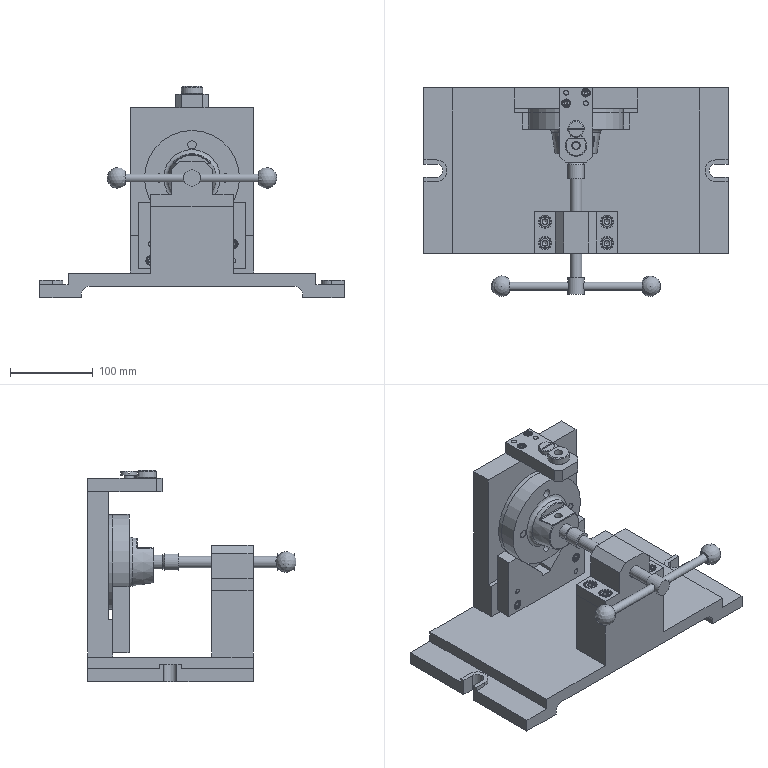Assembly | NX | mm | 27 component files | 27 solids | 499 faces | box 368 x 252.5 x 256 mm | volume 3203804 mm3 | plane 256 | cone 118 | cylinder 98 | torus 19 | sphere 4 | spline 4 | commonest cylinder face diameters 6 x15 10 x15 8 x12 15 x6 20 x5 9 x5 7.76 x4 13 x4
Bill of materials:
GB-T70.1-2000,M8x20 | 4 |  | Hexagon Socket Head Cap Screw, GB-T 70.1-2000,M8x20
unnamed part 1 | 1 |  | Long, slender cylindrical pin with a short, smaller-diameter stepped journal at each end.
unnamed part 2 | 1 |  | Cylindrical pin with a larger-diameter head at one end. A transverse through-hole crosses the head. The opposite end steps down to a short smaller-diameter journal.
unnamed part 3 | 1 |  | Stepped shaft: a hexagonal section at one end, a larger cylindrical collar in the middle, and a smaller cylindrical spigot with a chamfered end.
unnamed part 4 | 1 |  | Thick-walled cylindrical sleeve with a central bore and an outer chamfer at one end.
GB-T119.1-2000,10x30 | 1 |  | Parallel Pin, GB-T 119.1-2000,10x30
unnamed part 5 | 1 |  | Shouldered pin with a slotted head: a chamfered disc head with a straight slot, a cylindrical shoulder, a narrow neck or undercut, and a chamfered cylindrical pilot end.
unnamed part 6 | 1 |  | Pillow-block-style bracket: a rectangular base plate with a raised central block. The block has chamfered upper corners and one horizontal through-bore.
unnamed part 7 | 1 |  | Flanged bushing: a cylindrical body with a larger chamfered flange at one end and a central through-bore. The flange has a flat or notch cut on one side.
GB-T119.1-2000,6x22 | 2 |  | Parallel Pin, GB-T 119.1-2000,6x22
unnamed part 8 | 2 |  | Sphere with uniform, ball-like form.
unnamed part 9 | 1 |  | Plain cylindrical tube or spacer ring with a concentric through-bore and square ends.
unnamed part 10 | 1 |  | Rectangular plate with a symmetric V-shaped notch cut into one long edge. A small rectangular slot sits at the bottom of the V. The plate has four through-holes near its ends.
unnamed part 11 | 1 |  | Circular flange with a tapered hub on one side. The hub has a flat face with a cross-hole and ends in a small cylindrical spigot. The opposite face has a central circular recess.
unnamed part 12 | 1 |  | Rectangular plate with two chamfered corners at one end, one large through-hole, one medium hole, and four small holes grouped at the opposite end.
GB-T119.1-2000,6x26 | 2 |  | Parallel Pin, GB-T 119.1-2000,6x26
unnamed part 13 | 1 |  | Prismatic, machined-looking base plate with a rectangular block standing near one end and a tall upright plate near the other. The base has thinner stepped flanges at both ends, each with an open-ended U-slot, and a wide shallow relief with rounded ends across the underside. The upright plate has a slightly raised or recessed circular face carrying small holes, a raised strip along its lower edge with holes, and small holes on its top edge. The block has holes on its top face.
GB-T70.1-2000,M5x16 | 2 |  | Hexagon Socket Head Cap Screw, GB-T 70.1-2000,M5x16
GB-T70.1-2000,M6x20 | 2 |  | Hexagon Socket Head Cap Screw, GB-T 70.1-2000,M6x20
Mates:
1. fix | fixture_body 1 component
2. concentric | base 1 edge | fixture_body 1 edge
3. touch align | fixed_v_block 1 face | base 1 face
4. touch align | fixed_v_block 1 face | base 1 face
5. touch align | fixed_v_block 1 face | base 1 face
6. concentric | bushing 1 edge | drill_template 1 edge
7. concentric | drill_bushing 1 edge | bushing 1 edge
8. concentric | drill_bushing_screw 1 edge | drill_template 1 edge
9. touch align | drill_template 1 face | fixture_body 1 face
10. center | drill_template 1 face | drill_template 1 face | fixture_body 1 face | fixture_body 1 face
11. touch align | drill_template 1 face | fixture_body 1 face
12. touch align | screw_rod 1 face | fixed_bracket 1 face
13. concentric | rubber_pad 1 edge | screw_rod 1 edge
14. touch align | rubber_pad 1 face | base 1 face
15. touch align | handle 1 face | screw_rod 1 face
16. center | handle 1 face | handle 1 face | fixed_bracket 1 face | fixed_bracket 1 face
17. concentric | handle_1 2 edge | handle 1 edge
18. concentric | handle_1 1 edge | handle 1 edge
19. concentric | diamond_locating_pin 1 edge | fixture_body 1 edge
20. concentric | GB-T70_1-2000_M8x20 1 edge | fixed_bracket 1 edge
21. concentric | GB-T70_1-2000_M8x20 2 edge | fixed_bracket 1 edge
22. concentric | GB-T70_1-2000_M8x20 3 edge | fixed_bracket 1 edge
23. concentric | GB-T70_1-2000_M8x20 4 edge | fixed_bracket 1 edge
24. concentric | GB-T119_1-2000_6x22 1 edge | drill_template 1 edge
25. concentric | GB-T119_1-2000_6x22 2 edge | drill_template 1 edge
26. concentric | GB-T70_1-2000_M5x16 2 edge | drill_template 1 edge
27. concentric | GB-T70_1-2000_M5x16 1 edge | drill_template 1 edge
28. concentric | GB-T70_1-2000_M6x20 2 edge | fixed_v_block 1 edge
29. concentric | GB-T70_1-2000_M6x20 1 edge | fixed_v_block 1 edge
30. concentric | GB-T119_1-2000_6x26 2 edge | fixed_v_block 1 edge
31. concentric | GB-T119_1-2000_6x26 1 edge | fixed_v_block 1 edge